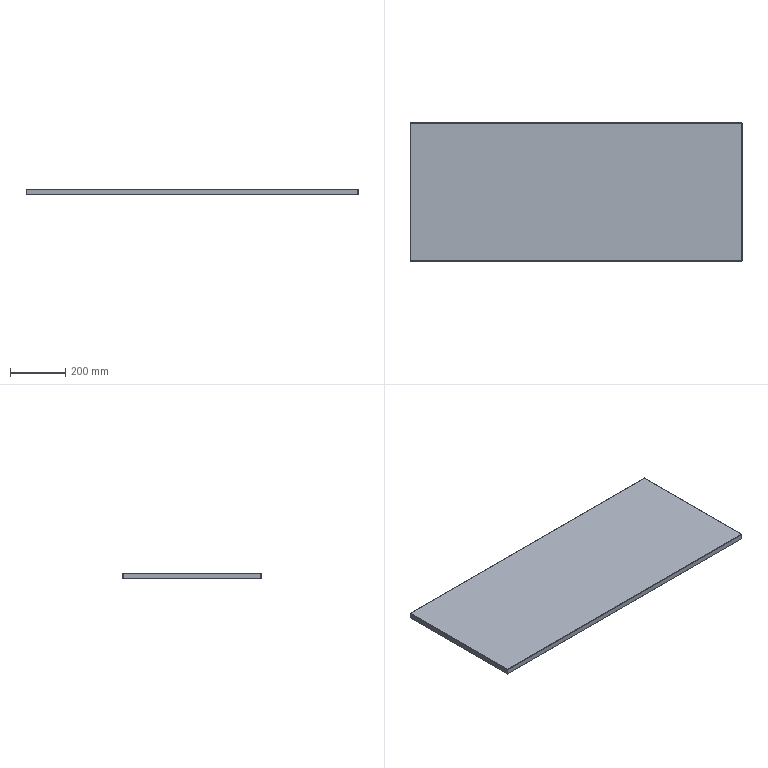Component | SolidWorks | TopPlate-1_TopPanelOuterPanel-1 | 1 solid | 38 faces | volume 530402 mm3 | plane 22 | spline 8 | cylinder 8 | commonest cylinder face diameters 3.6 x4 2 x4 | material 304